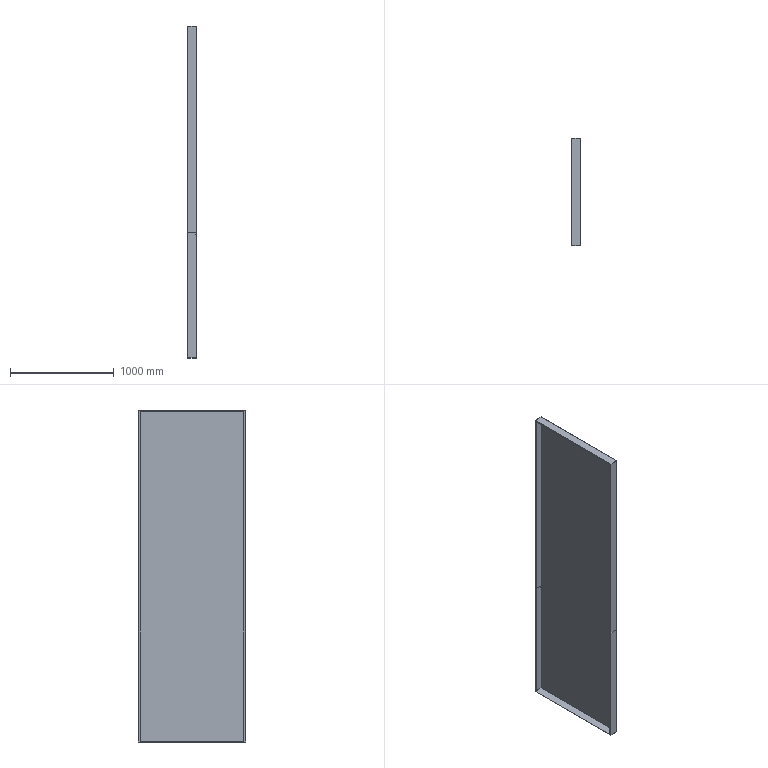Component | NX | CB1 | 1 solid | 30 faces | volume 6079585 mm3 | plane 30